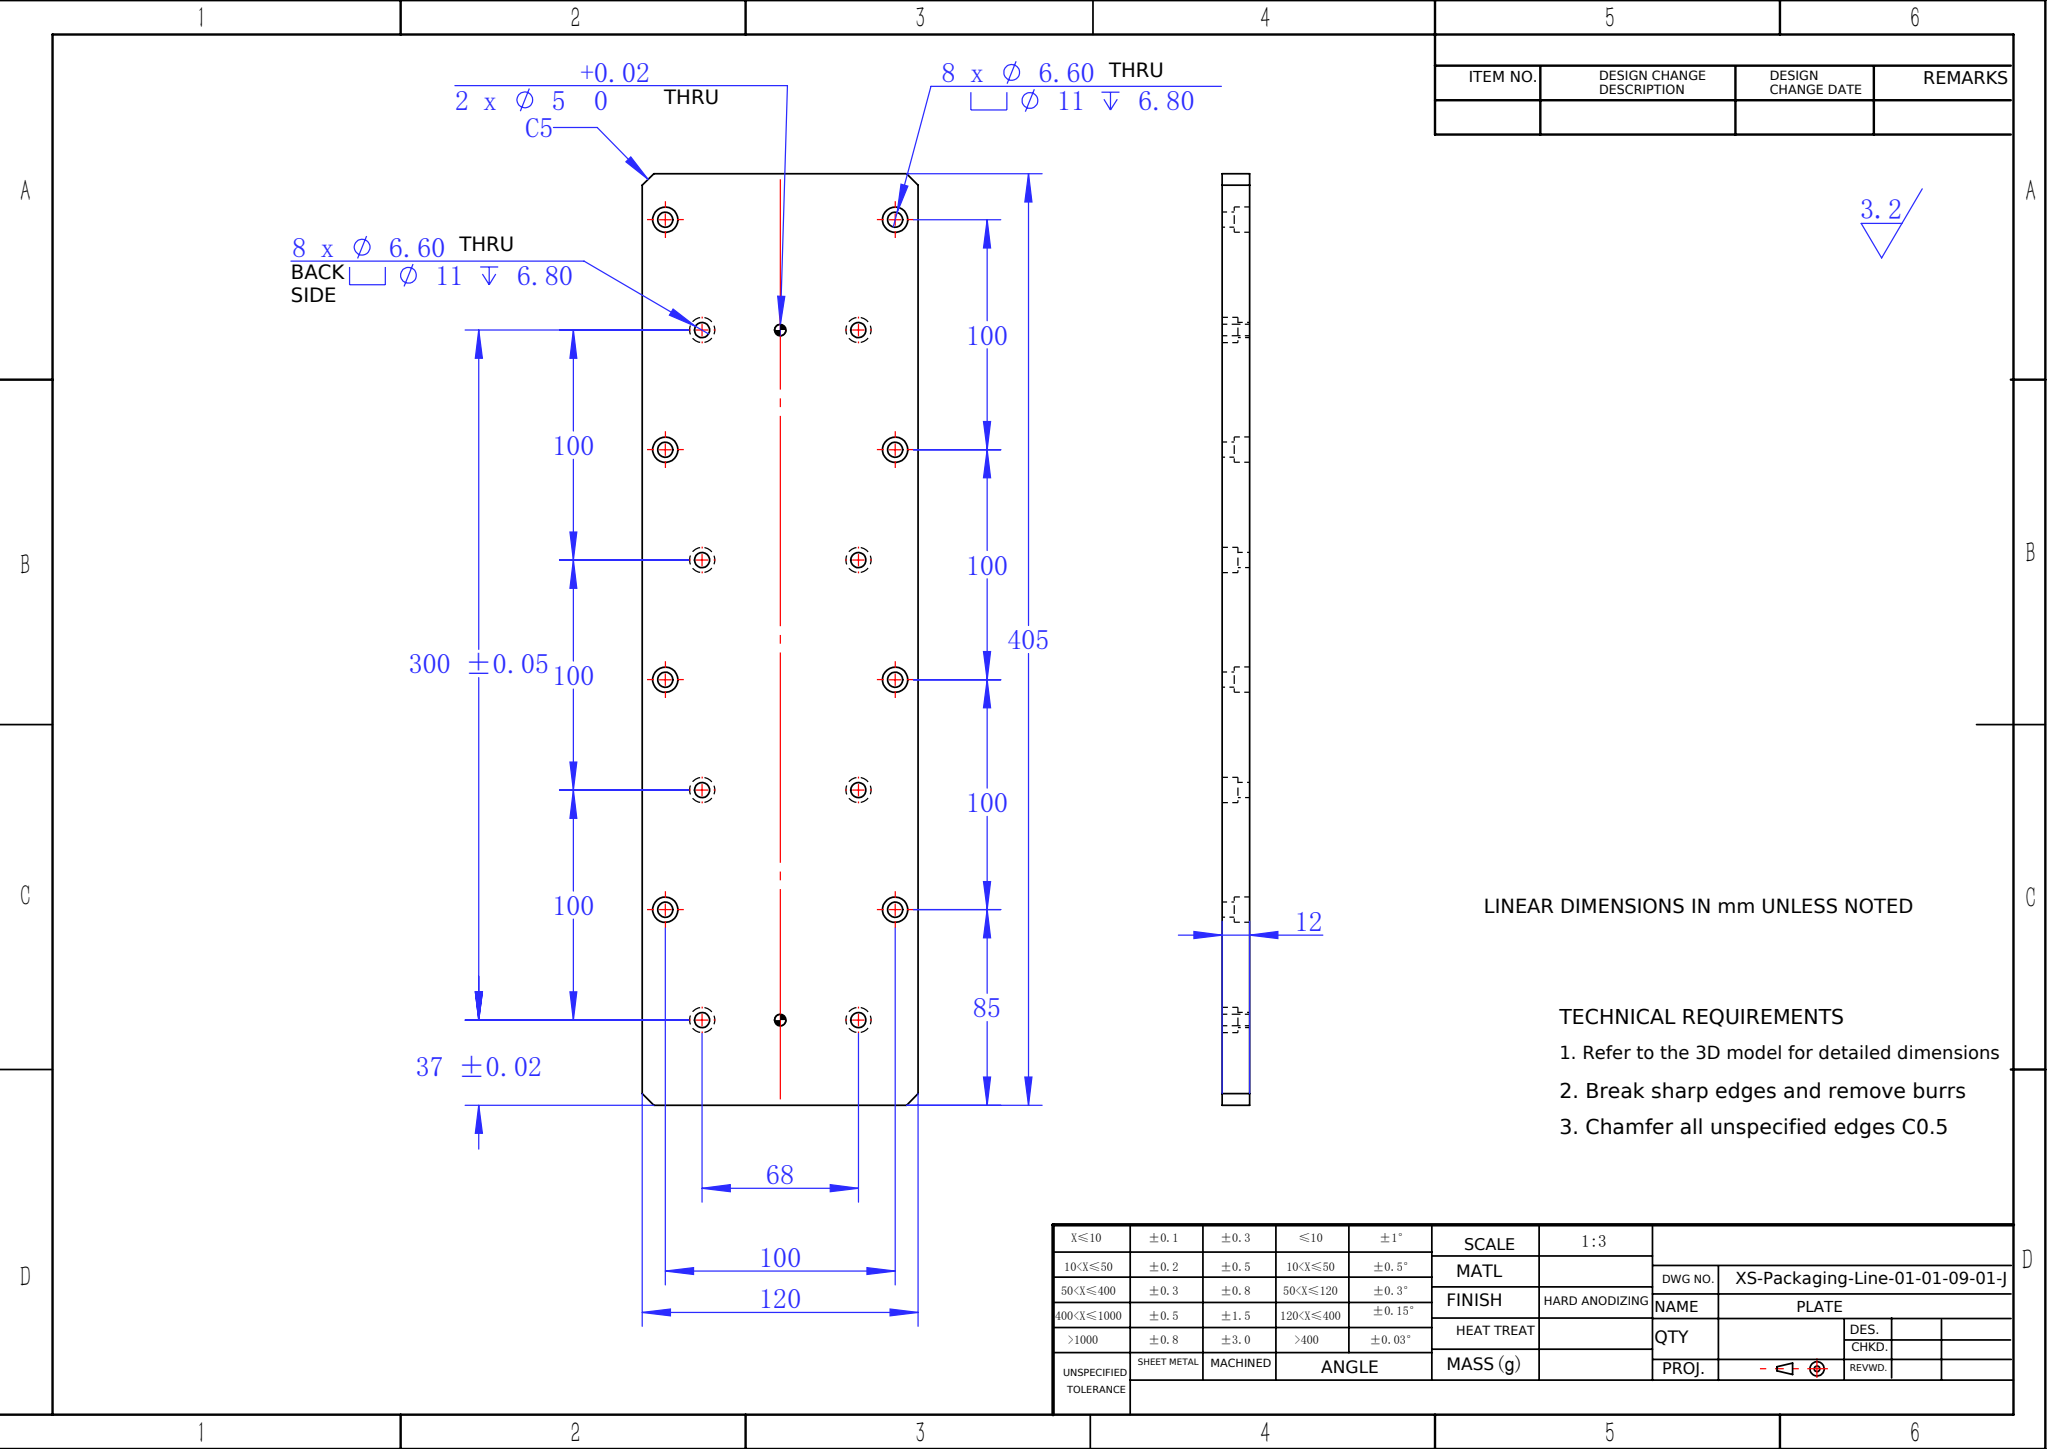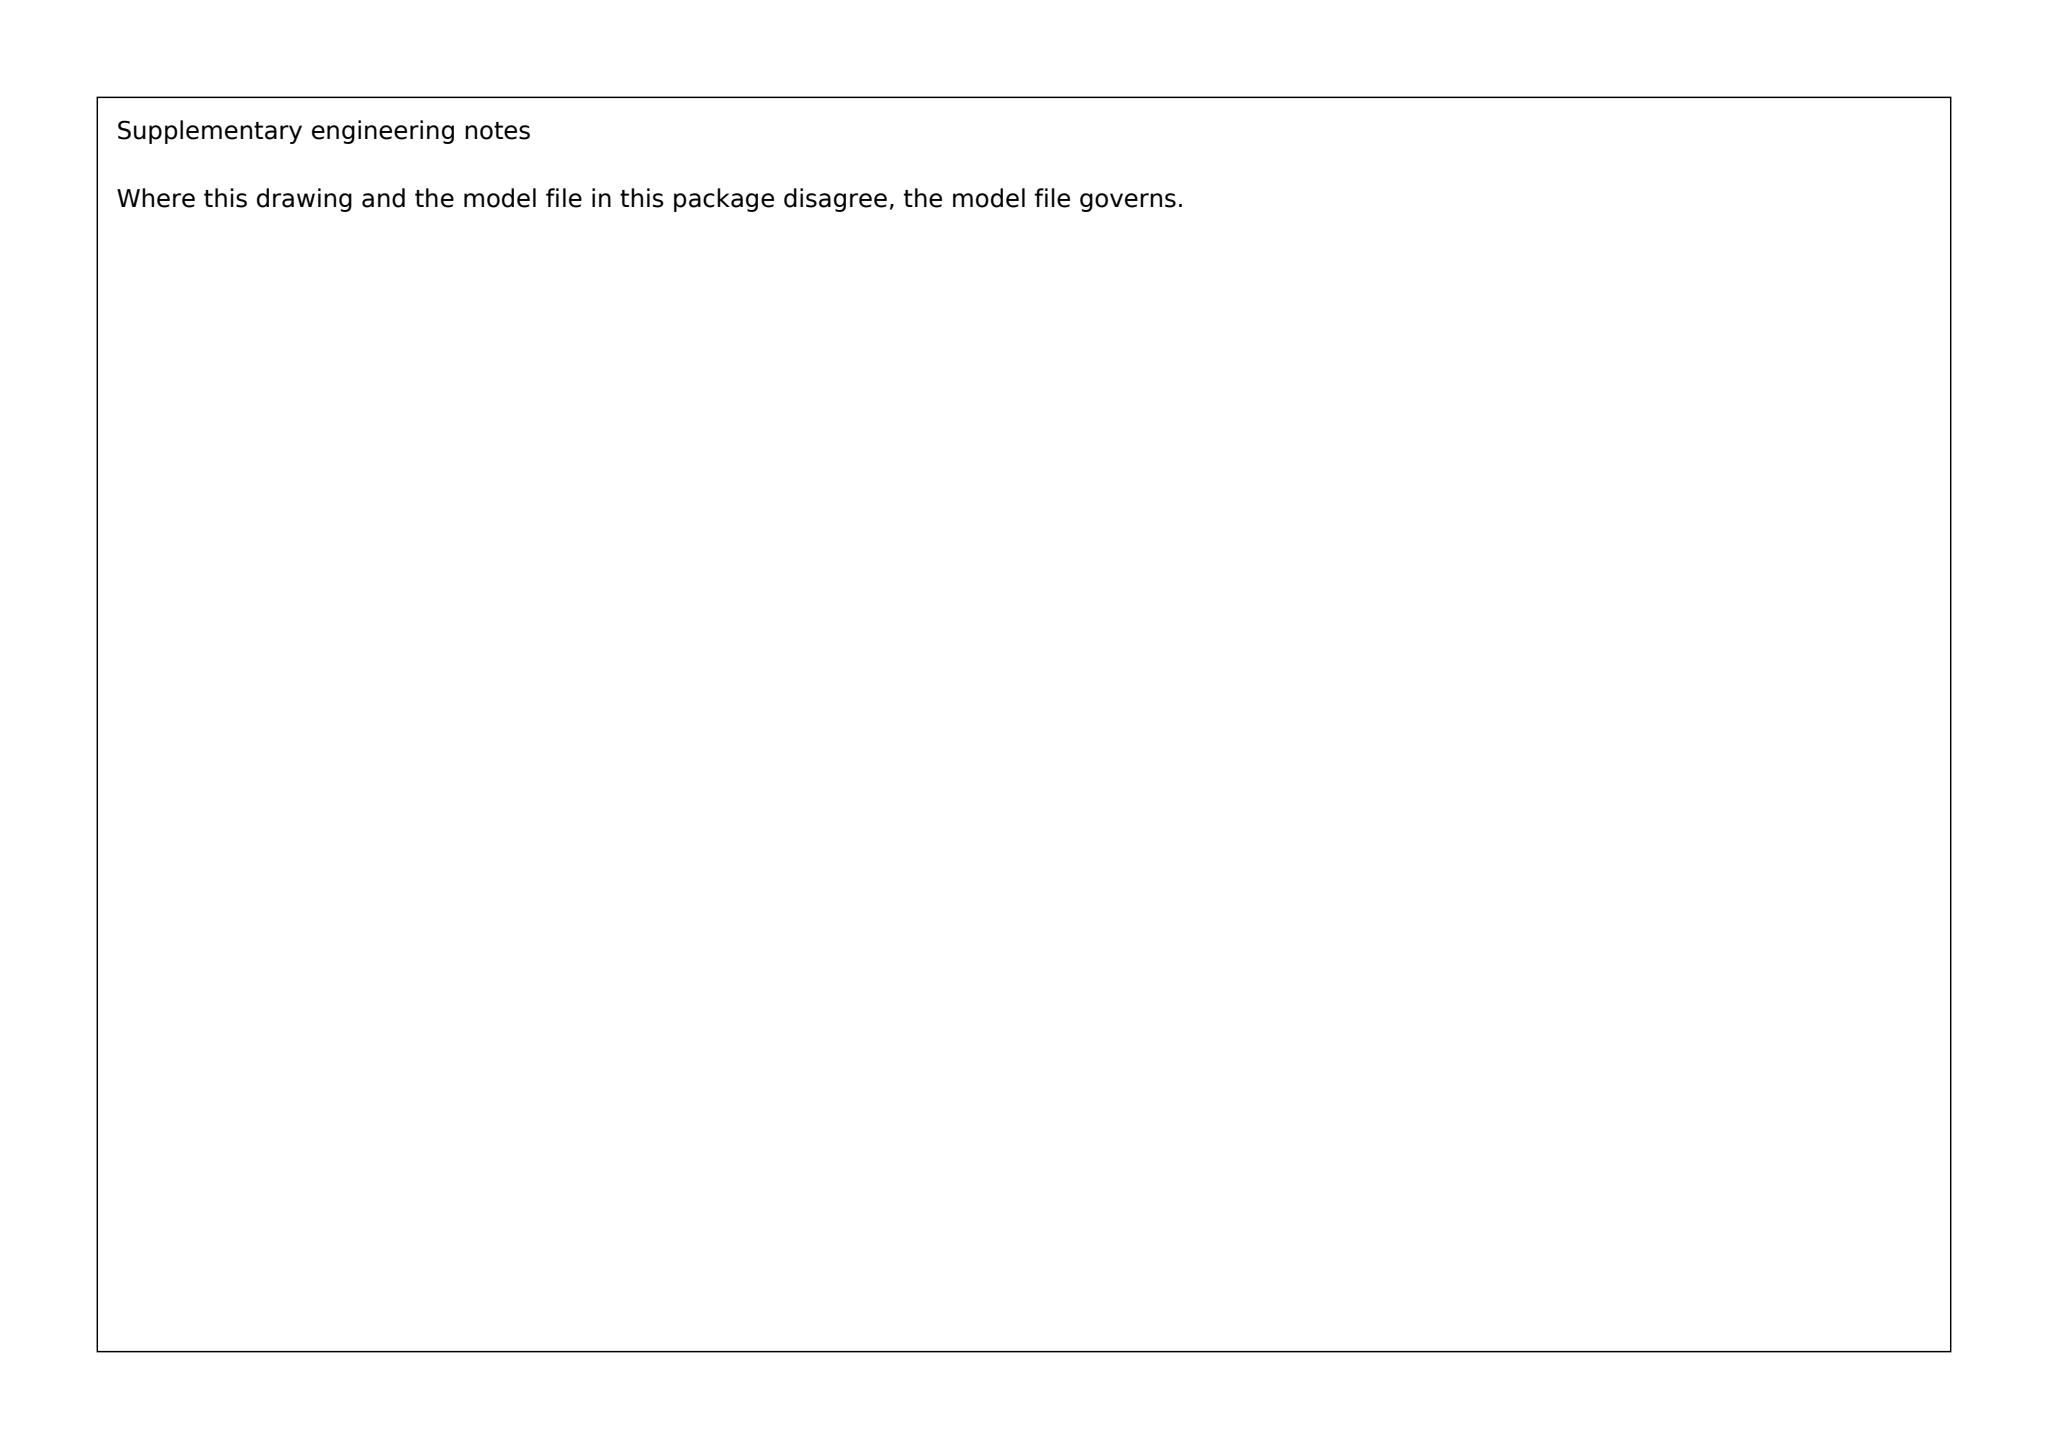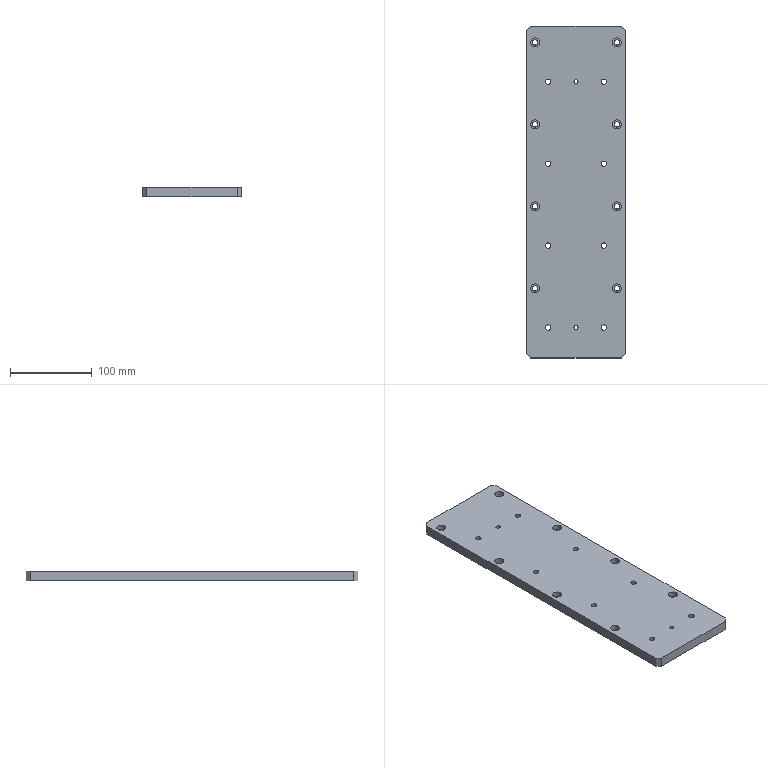Part | SolidWorks | mm | 1 solid | 94 faces | box 120 x 405 x 12 mm | volume 568943 mm3 | cylinder 68 | plane 26 | commonest cylinder face diameters 11 x32 6.6 x32 5 x4
build123d program:
from build123d import *

# Parameters (mm, degrees)
SKETCH1_W                                       = 120
SKETCH1_H                                       = 405
BOSS_EXTRUDE1_DEPTH                             = 12
M6_HEX_SOCKET_HEAD_CAP_SCREW_CBORE1_D           = 6.6
M6_HEX_SOCKET_HEAD_CAP_SCREW_CBORE1_CBORE_D     = 11
M6_HEX_SOCKET_HEAD_CAP_SCREW_CBORE1_CBORE_DEPTH = 6.8
CHAMFER1_SIZE                                   = 5
M6_HEX_SOCKET_HEAD_CAP_SCREW_CBORE2_D           = 6.6
M6_HEX_SOCKET_HEAD_CAP_SCREW_CBORE2_CBORE_D     = 11
M6_HEX_SOCKET_HEAD_CAP_SCREW_CBORE2_CBORE_DEPTH = 6.8
F_5_0MM_DOWEL_PIN_HOLE1_D                       = 5
LPATTERN1_COUNT                                 = 2
LPATTERN1_PITCH                                 = 300


with BuildPart() as part:
    # Sketch1 → Boss-Extrude1 (new body)
    with BuildSketch(Plane.XY):
        Rectangle(SKETCH1_W, SKETCH1_H)
    extrude(amount=BOSS_EXTRUDE1_DEPTH)

    # M6 Hex Socket Head Cap Screw CBORE1 (through all)
    with Locations(Plane.XY.offset(12)):
        with Locations((-50, 182.5), (50, 182.5), (-50, 82.5), (50, 82.5), (-50, -17.5), (50, -17.5), (-50, -117.5), (50, -117.5)):
            CounterBoreHole(M6_HEX_SOCKET_HEAD_CAP_SCREW_CBORE1_D / 2, M6_HEX_SOCKET_HEAD_CAP_SCREW_CBORE1_CBORE_D / 2, M6_HEX_SOCKET_HEAD_CAP_SCREW_CBORE1_CBORE_DEPTH)

    # Chamfer1
    chamfer1_edges = [part.edges().sort_by_distance(p)[0] for p in [
        (60, -202.5, 6),
        (-60, -202.5, 6),
        (-60, 202.5, 6),
        (60, 202.5, 6),
    ]]
    chamfer(chamfer1_edges, length=CHAMFER1_SIZE)

    # M6 Hex Socket Head Cap Screw CBORE2 (through all)
    with Locations(Plane(origin=(0, 0, 0), x_dir=(-1, 0, 0), z_dir=(0, 0, -1))):
        with Locations((-34, -165.5), (-34, 134.5), (-34, -65.5), (-34, 34.5), (34, 134.5), (34, 34.5), (34, -65.5), (34, -165.5)):
            CounterBoreHole(M6_HEX_SOCKET_HEAD_CAP_SCREW_CBORE2_D / 2, M6_HEX_SOCKET_HEAD_CAP_SCREW_CBORE2_CBORE_D / 2, M6_HEX_SOCKET_HEAD_CAP_SCREW_CBORE2_CBORE_DEPTH)

    # 5.0mm Dowel Pin Hole1 (through all)
    with Locations(Plane(origin=(0, 0, 0), x_dir=(-1, 0, 0), z_dir=(0, 0, -1))):
        with Locations((0, -165.5)):
            f_5_0mm_dowel_pin_hole1 = Hole(F_5_0MM_DOWEL_PIN_HOLE1_D / 2)

    # LPattern1: 5.0mm Dowel Pin Hole1 ×2
    with Locations(*[(0, i * LPATTERN1_PITCH, 0) for i in range(1, LPATTERN1_COUNT)]):
        add(f_5_0mm_dowel_pin_hole1, mode=Mode.SUBTRACT)


solid = part.part